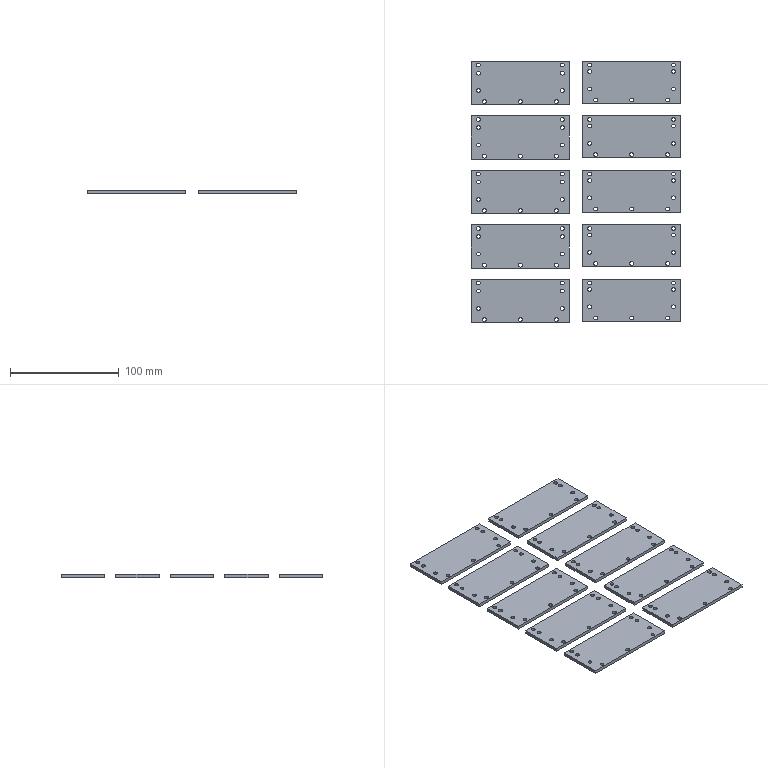CAM job | Mastercam | mm | 4 operations | part box 192.08 x 240.3 x 3
1. Contour (Ramp) | 4 - 4 平铣刀
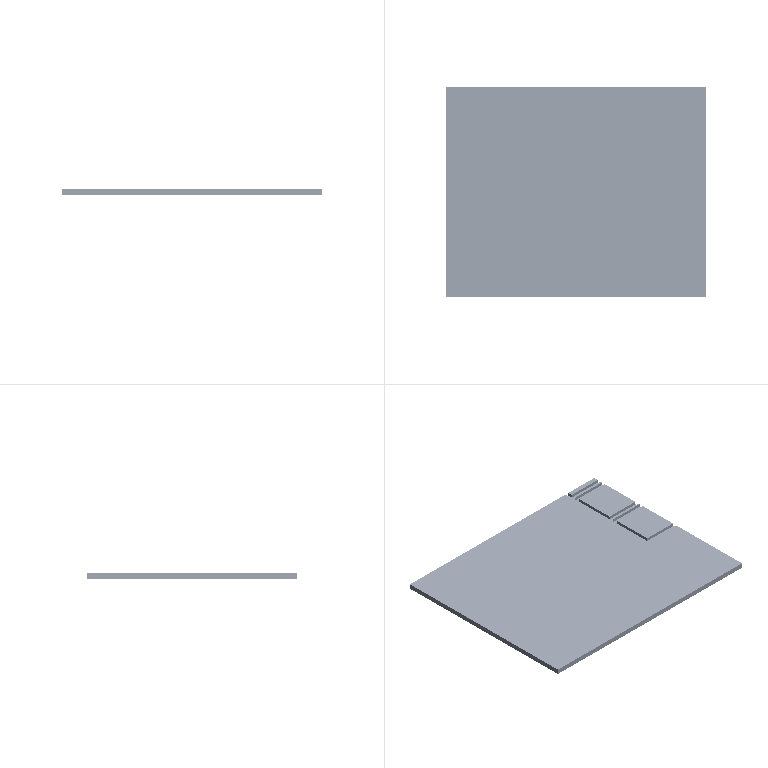2. Drill/Counterbore | 5 - 4 倒角刀
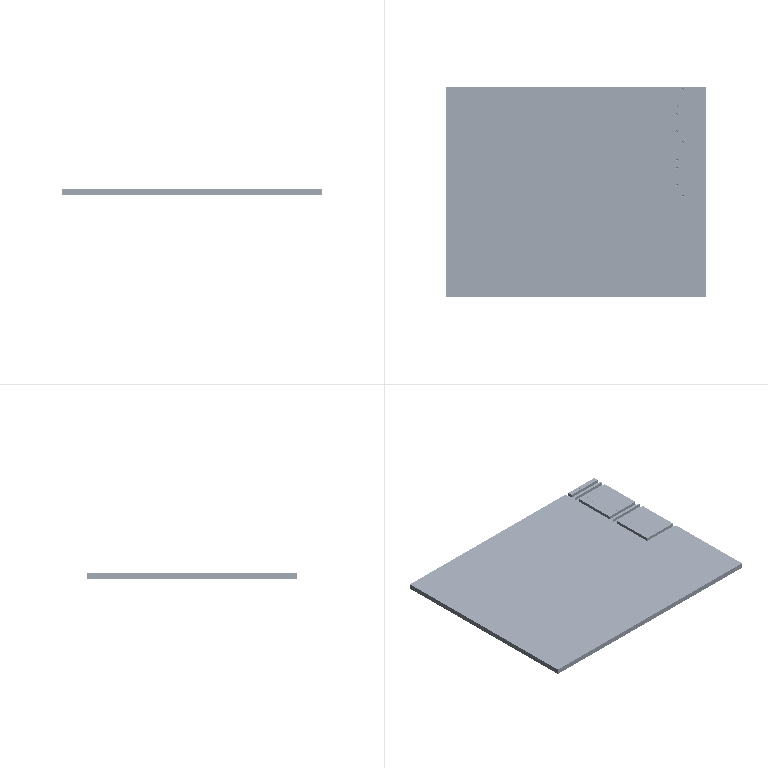3. Contour (2D chamfer) | 5 - 4 倒角刀
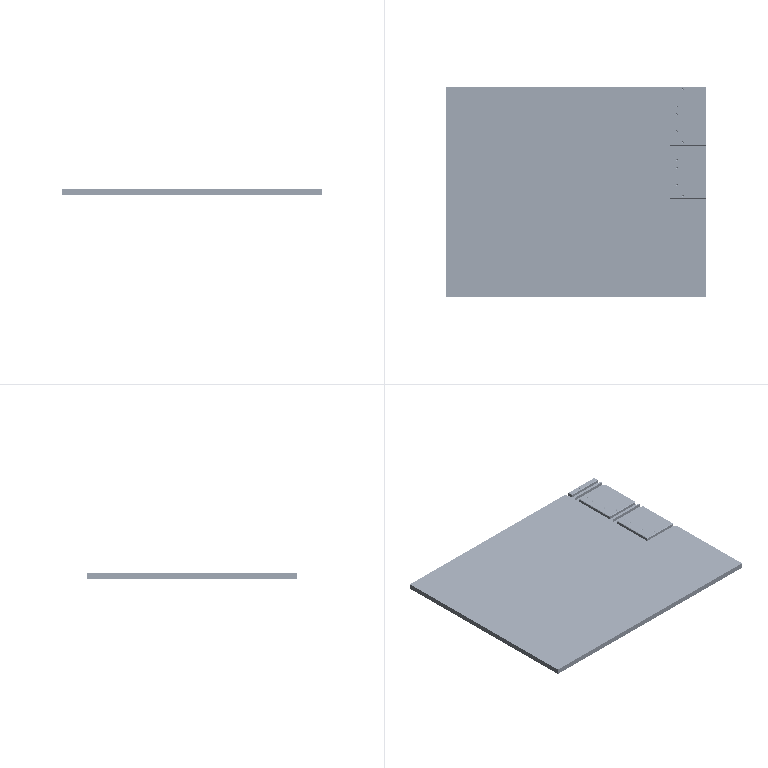4. Contour (2D) | 3 - 3 平铣刀